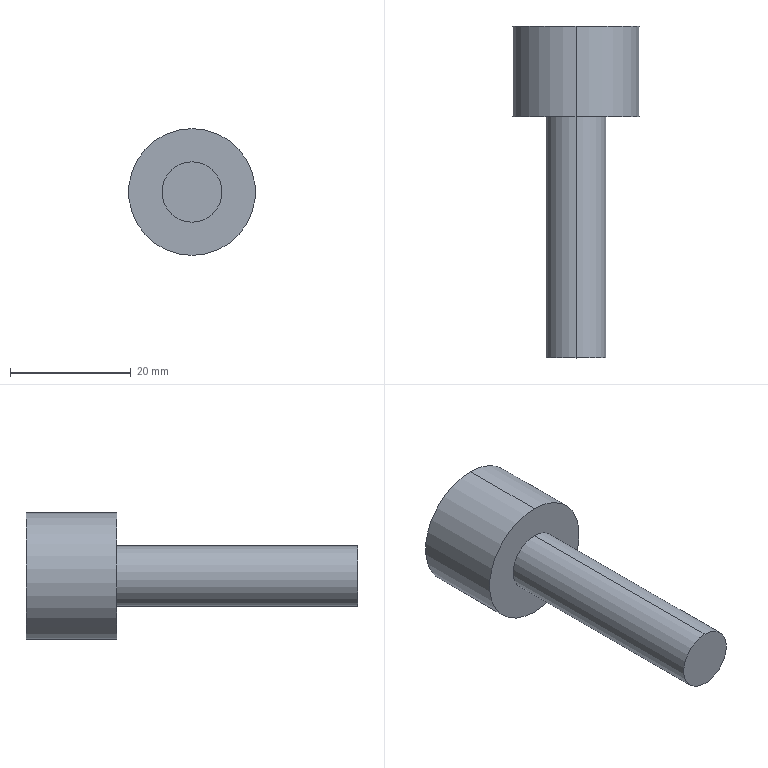Component | SolidWorks | SpringPullPlateFixingAxis-1 | 1 solid | 7 faces | box 21 x 55 x 21 mm | volume 8337 mm3 | cylinder 4 | plane 3 | commonest cylinder face diameters 10 x2 21 x2
build123d program:
from build123d import *


with BuildPart() as part:
    # Sketch1 → Revolve1 (revolve)
    with BuildSketch(Plane.XY, mode=Mode.PRIVATE) as revolve1_sk:
        Polygon((0, 29.928), (10.5, 29.928), (10.5, 14.928), (5, 14.928), (5, -25.072), (0, -25.072), align=None)
    revolve(revolve1_sk.sketch.rotate(Axis((0, 0, 0), (0, 1, 0)), 90), axis=Axis((0, 0, 0), (0, 1, 0)))


solid = part.part

# Placed as in the assembly
solid = solid.moved(Location((250.216, 400.055, -208.5), (0, 0, 0)))
STEP:
#1=COLOUR_RGB('',0.7922,0.8196,0.9333);
#2=FILL_AREA_STYLE_COLOUR('',#1);
#3=FILL_AREA_STYLE('',(#2));
#4=SURFACE_STYLE_FILL_AREA(#3);
#5=SURFACE_SIDE_STYLE('',(#4));
#6=SURFACE_STYLE_USAGE(.BOTH.,#5);
#7=PRESENTATION_STYLE_ASSIGNMENT((#6));
#8=CARTESIAN_POINT('',(9.851,16.338,-8.406));
#9=VERTEX_POINT('',#8);
#10=CARTESIAN_POINT('',(9.851,16.338,-8.012));
#11=VERTEX_POINT('',#10);
#12=CARTESIAN_POINT('',(9.851,16.338,-8.209));
#13=DIRECTION('',(0.,-1.,0.));
#14=DIRECTION('',(0.,0.,-1.));
#15=AXIS2_PLACEMENT_3D('',#12,#13,#14);
#16=CIRCLE('',#15,0.1969);
#17=EDGE_CURVE('',#9,#11,#16,.T.);
#18=ORIENTED_EDGE('',*,*,#17,.T.);
#19=CARTESIAN_POINT('',(9.851,14.763,-8.012));
#20=VERTEX_POINT('',#19);
#21=CARTESIAN_POINT('',(9.851,15.75,-8.012));
#22=DIRECTION('',(0.,-1.,0.));
#23=VECTOR('',#22,39.37);
#24=LINE('',#21,#23);
#25=EDGE_CURVE('',#11,#20,#24,.T.);
#26=ORIENTED_EDGE('',*,*,#25,.T.);
#27=CARTESIAN_POINT('',(9.851,14.763,-8.406));
#28=VERTEX_POINT('',#27);
#29=CARTESIAN_POINT('',(9.851,14.763,-8.209));
#30=DIRECTION('',(0.,-1.,0.));
#31=DIRECTION('',(0.,0.,-1.));
#32=AXIS2_PLACEMENT_3D('',#29,#30,#31);
#33=CIRCLE('',#32,0.1969);
#34=EDGE_CURVE('',#28,#20,#33,.T.);
#35=ORIENTED_EDGE('',*,*,#34,.F.);
#36=CARTESIAN_POINT('',(9.851,15.75,-8.406));
#37=DIRECTION('',(0.,-1.,0.));
#38=VECTOR('',#37,39.37);
#39=LINE('',#36,#38);
#40=EDGE_CURVE('',#9,#28,#39,.T.);
#41=ORIENTED_EDGE('',*,*,#40,.F.);
#42=EDGE_LOOP('',(#18,#26,#35,#41));
#43=FACE_OUTER_BOUND('',#42,.T.);
#44=CARTESIAN_POINT('',(9.851,15.75,-8.209));
#45=DIRECTION('',(0.,-1.,0.));
#46=DIRECTION('',(0.,0.,-1.));
#47=AXIS2_PLACEMENT_3D('',#44,#45,#46);
#48=CYLINDRICAL_SURFACE('',#47,0.1969);
#49=ADVANCED_FACE('',(#43),#48,.T.);
#50=CARTESIAN_POINT('',(9.851,16.928,-8.622));
#51=VERTEX_POINT('',#50);
#52=CARTESIAN_POINT('',(9.851,16.928,-7.795));
#53=VERTEX_POINT('',#52);
#54=CARTESIAN_POINT('',(9.851,16.928,-8.209));
#55=DIRECTION('',(0.,-1.,0.));
#56=DIRECTION('',(0.,0.,-1.));
#57=AXIS2_PLACEMENT_3D('',#54,#55,#56);
#58=CIRCLE('',#57,0.4134);
#59=EDGE_CURVE('',#51,#53,#58,.T.);
#60=ORIENTED_EDGE('',*,*,#59,.T.);
#61=CARTESIAN_POINT('',(9.851,16.338,-7.795));
#62=VERTEX_POINT('',#61);
#63=CARTESIAN_POINT('',(9.851,15.75,-7.795));
#64=DIRECTION('',(0.,-1.,0.));
#65=VECTOR('',#64,39.37);
#66=LINE('',#63,#65);
#67=EDGE_CURVE('',#53,#62,#66,.T.);
#68=ORIENTED_EDGE('',*,*,#67,.T.);
#69=CARTESIAN_POINT('',(9.851,16.338,-8.622));
#70=VERTEX_POINT('',#69);
#71=CARTESIAN_POINT('',(9.851,16.338,-8.209));
#72=DIRECTION('',(0.,-1.,0.));
#73=DIRECTION('',(0.,0.,-1.));
#74=AXIS2_PLACEMENT_3D('',#71,#72,#73);
#75=CIRCLE('',#74,0.4134);
#76=EDGE_CURVE('',#70,#62,#75,.T.);
#77=ORIENTED_EDGE('',*,*,#76,.F.);
#78=CARTESIAN_POINT('',(9.851,15.75,-8.622));
#79=DIRECTION('',(0.,-1.,0.));
#80=VECTOR('',#79,39.37);
#81=LINE('',#78,#80);
#82=EDGE_CURVE('',#51,#70,#81,.T.);
#83=ORIENTED_EDGE('',*,*,#82,.F.);
#84=EDGE_LOOP('',(#60,#68,#77,#83));
#85=FACE_OUTER_BOUND('',#84,.T.);
#86=CARTESIAN_POINT('',(9.851,15.75,-8.209));
#87=DIRECTION('',(0.,-1.,0.));
#88=DIRECTION('',(0.,0.,-1.));
#89=AXIS2_PLACEMENT_3D('',#86,#87,#88);
#90=CYLINDRICAL_SURFACE('',#89,0.4134);
#91=ADVANCED_FACE('',(#85),#90,.T.);
#92=ORIENTED_EDGE('',*,*,#59,.F.);
#93=CARTESIAN_POINT('',(9.851,16.928,-8.209));
#94=DIRECTION('',(0.,-1.,0.));
#95=DIRECTION('',(0.,0.,-1.));
#96=AXIS2_PLACEMENT_3D('',#93,#94,#95);
#97=CIRCLE('',#96,0.4134);
#98=EDGE_CURVE('',#53,#51,#97,.T.);
#99=ORIENTED_EDGE('',*,*,#98,.F.);
#100=EDGE_LOOP('',(#92,#99));
#101=FACE_OUTER_BOUND('',#100,.T.);
#102=CARTESIAN_POINT('',(9.851,16.928,-8.209));
#103=DIRECTION('',(0.,1.,0.));
#104=DIRECTION('',(0.,0.,1.));
#105=AXIS2_PLACEMENT_3D('',#102,#103,#104);
#106=PLANE('',#105);
#107=ADVANCED_FACE('',(#101),#106,.T.);
#108=ORIENTED_EDGE('',*,*,#67,.F.);
#109=ORIENTED_EDGE('',*,*,#98,.T.);
#110=ORIENTED_EDGE('',*,*,#82,.T.);
#111=CARTESIAN_POINT('',(9.851,16.338,-8.209));
#112=DIRECTION('',(0.,-1.,0.));
#113=DIRECTION('',(0.,0.,-1.));
#114=AXIS2_PLACEMENT_3D('',#111,#112,#113);
#115=CIRCLE('',#114,0.4134);
#116=EDGE_CURVE('',#62,#70,#115,.T.);
#117=ORIENTED_EDGE('',*,*,#116,.F.);
#118=EDGE_LOOP('',(#108,#109,#110,#117));
#119=FACE_OUTER_BOUND('',#118,.T.);
#120=CARTESIAN_POINT('',(9.851,15.75,-8.209));
#121=DIRECTION('',(0.,-1.,0.));
#122=DIRECTION('',(0.,0.,-1.));
#123=AXIS2_PLACEMENT_3D('',#120,#121,#122);
#124=CYLINDRICAL_SURFACE('',#123,0.4134);
#125=ADVANCED_FACE('',(#119),#124,.T.);
#126=ORIENTED_EDGE('',*,*,#76,.T.);
#127=ORIENTED_EDGE('',*,*,#116,.T.);
#128=EDGE_LOOP('',(#126,#127));
#129=FACE_OUTER_BOUND('',#128,.T.);
#130=ORIENTED_EDGE('',*,*,#17,.F.);
#131=CARTESIAN_POINT('',(9.851,16.338,-8.209));
#132=DIRECTION('',(0.,-1.,0.));
#133=DIRECTION('',(0.,0.,-1.));
#134=AXIS2_PLACEMENT_3D('',#131,#132,#133);
#135=CIRCLE('',#134,0.1969);
#136=EDGE_CURVE('',#11,#9,#135,.T.);
#137=ORIENTED_EDGE('',*,*,#136,.F.);
#138=EDGE_LOOP('',(#130,#137));
#139=FACE_BOUND('',#138,.T.);
#140=CARTESIAN_POINT('',(10.264,16.338,-8.209));
#141=DIRECTION('',(0.,-1.,0.));
#142=DIRECTION('',(0.,0.,-1.));
#143=AXIS2_PLACEMENT_3D('',#140,#141,#142);
#144=PLANE('',#143);
#145=ADVANCED_FACE('',(#129,#139),#144,.T.);
#146=ORIENTED_EDGE('',*,*,#25,.F.);
#147=ORIENTED_EDGE('',*,*,#136,.T.);
#148=ORIENTED_EDGE('',*,*,#40,.T.);
#149=CARTESIAN_POINT('',(9.851,14.763,-8.209));
#150=DIRECTION('',(0.,-1.,0.));
#151=DIRECTION('',(0.,0.,-1.));
#152=AXIS2_PLACEMENT_3D('',#149,#150,#151);
#153=CIRCLE('',#152,0.1969);
#154=EDGE_CURVE('',#20,#28,#153,.T.);
#155=ORIENTED_EDGE('',*,*,#154,.F.);
#156=EDGE_LOOP('',(#146,#147,#148,#155));
#157=FACE_OUTER_BOUND('',#156,.T.);
#158=CARTESIAN_POINT('',(9.851,15.75,-8.209));
#159=DIRECTION('',(0.,-1.,0.));
#160=DIRECTION('',(0.,0.,-1.));
#161=AXIS2_PLACEMENT_3D('',#158,#159,#160);
#162=CYLINDRICAL_SURFACE('',#161,0.1969);
#163=ADVANCED_FACE('',(#157),#162,.T.);
#164=ORIENTED_EDGE('',*,*,#34,.T.);
#165=ORIENTED_EDGE('',*,*,#154,.T.);
#166=EDGE_LOOP('',(#164,#165));
#167=FACE_OUTER_BOUND('',#166,.T.);
#168=CARTESIAN_POINT('',(10.048,14.763,-8.209));
#169=DIRECTION('',(0.,-1.,0.));
#170=DIRECTION('',(0.,0.,-1.));
#171=AXIS2_PLACEMENT_3D('',#168,#169,#170);
#172=PLANE('',#171);
#173=ADVANCED_FACE('',(#167),#172,.T.);
#174=CLOSED_SHELL('',(#49,#91,#107,#125,#145,#163,#173));
#175=MANIFOLD_SOLID_BREP('',#174);
#176=STYLED_ITEM('',(#7),#175);
#177=PRESENTATION_LAYER_ASSIGNMENT('','',(#176));
#178=CARTESIAN_POINT('',(0.,0.,0.));
#179=DIRECTION('',(0.,0.,1.));
#180=DIRECTION('',(1.,0.,0.));
#181=AXIS2_PLACEMENT_3D('',#178,#179,#180);
#182=(LENGTH_UNIT()NAMED_UNIT(*)SI_UNIT($,.METRE.));
#183=LENGTH_MEASURE_WITH_UNIT(LENGTH_MEASURE(0.0254),#182);
#184=DIMENSIONAL_EXPONENTS(1.,0.,0.,0.,0.,0.,0.);
#185=(CONVERSION_BASED_UNIT('',#183)LENGTH_UNIT()NAMED_UNIT(#184));
#186=UNCERTAINTY_MEASURE_WITH_UNIT(LENGTH_MEASURE(0.00001),#185,'','');
#187=(NAMED_UNIT(*)PLANE_ANGLE_UNIT()SI_UNIT($,.RADIAN.));
#188=(NAMED_UNIT(*)SI_UNIT($,.STERADIAN.)SOLID_ANGLE_UNIT());
#189=(GEOMETRIC_REPRESENTATION_CONTEXT(3)GLOBAL_UNCERTAINTY_ASSIGNED_CONTEXT((#186))GLOBAL_UNIT_ASSIGNED_CONTEXT((#185,#187,#188))REPRESENTATION_CONTEXT('',''));
#190=ADVANCED_BREP_SHAPE_REPRESENTATION('',(#175,#181),#189);
#191=(LENGTH_UNIT()NAMED_UNIT(*)SI_UNIT($,.METRE.));
#192=LENGTH_MEASURE_WITH_UNIT(LENGTH_MEASURE(0.0254),#191);
#193=DIMENSIONAL_EXPONENTS(1.,0.,0.,0.,0.,0.,0.);
#194=(CONVERSION_BASED_UNIT('',#192)LENGTH_UNIT()NAMED_UNIT(#193));
#195=UNCERTAINTY_MEASURE_WITH_UNIT(LENGTH_MEASURE(0.00001),#194,'','');
#196=(NAMED_UNIT(*)PLANE_ANGLE_UNIT()SI_UNIT($,.RADIAN.));
#197=(NAMED_UNIT(*)SI_UNIT($,.STERADIAN.)SOLID_ANGLE_UNIT());
#198=(GEOMETRIC_REPRESENTATION_CONTEXT(3)GLOBAL_UNCERTAINTY_ASSIGNED_CONTEXT((#195))GLOBAL_UNIT_ASSIGNED_CONTEXT((#194,#196,#197))REPRESENTATION_CONTEXT('',''));
#199=MECHANICAL_DESIGN_GEOMETRIC_PRESENTATION_REPRESENTATION('',(#176),#198);